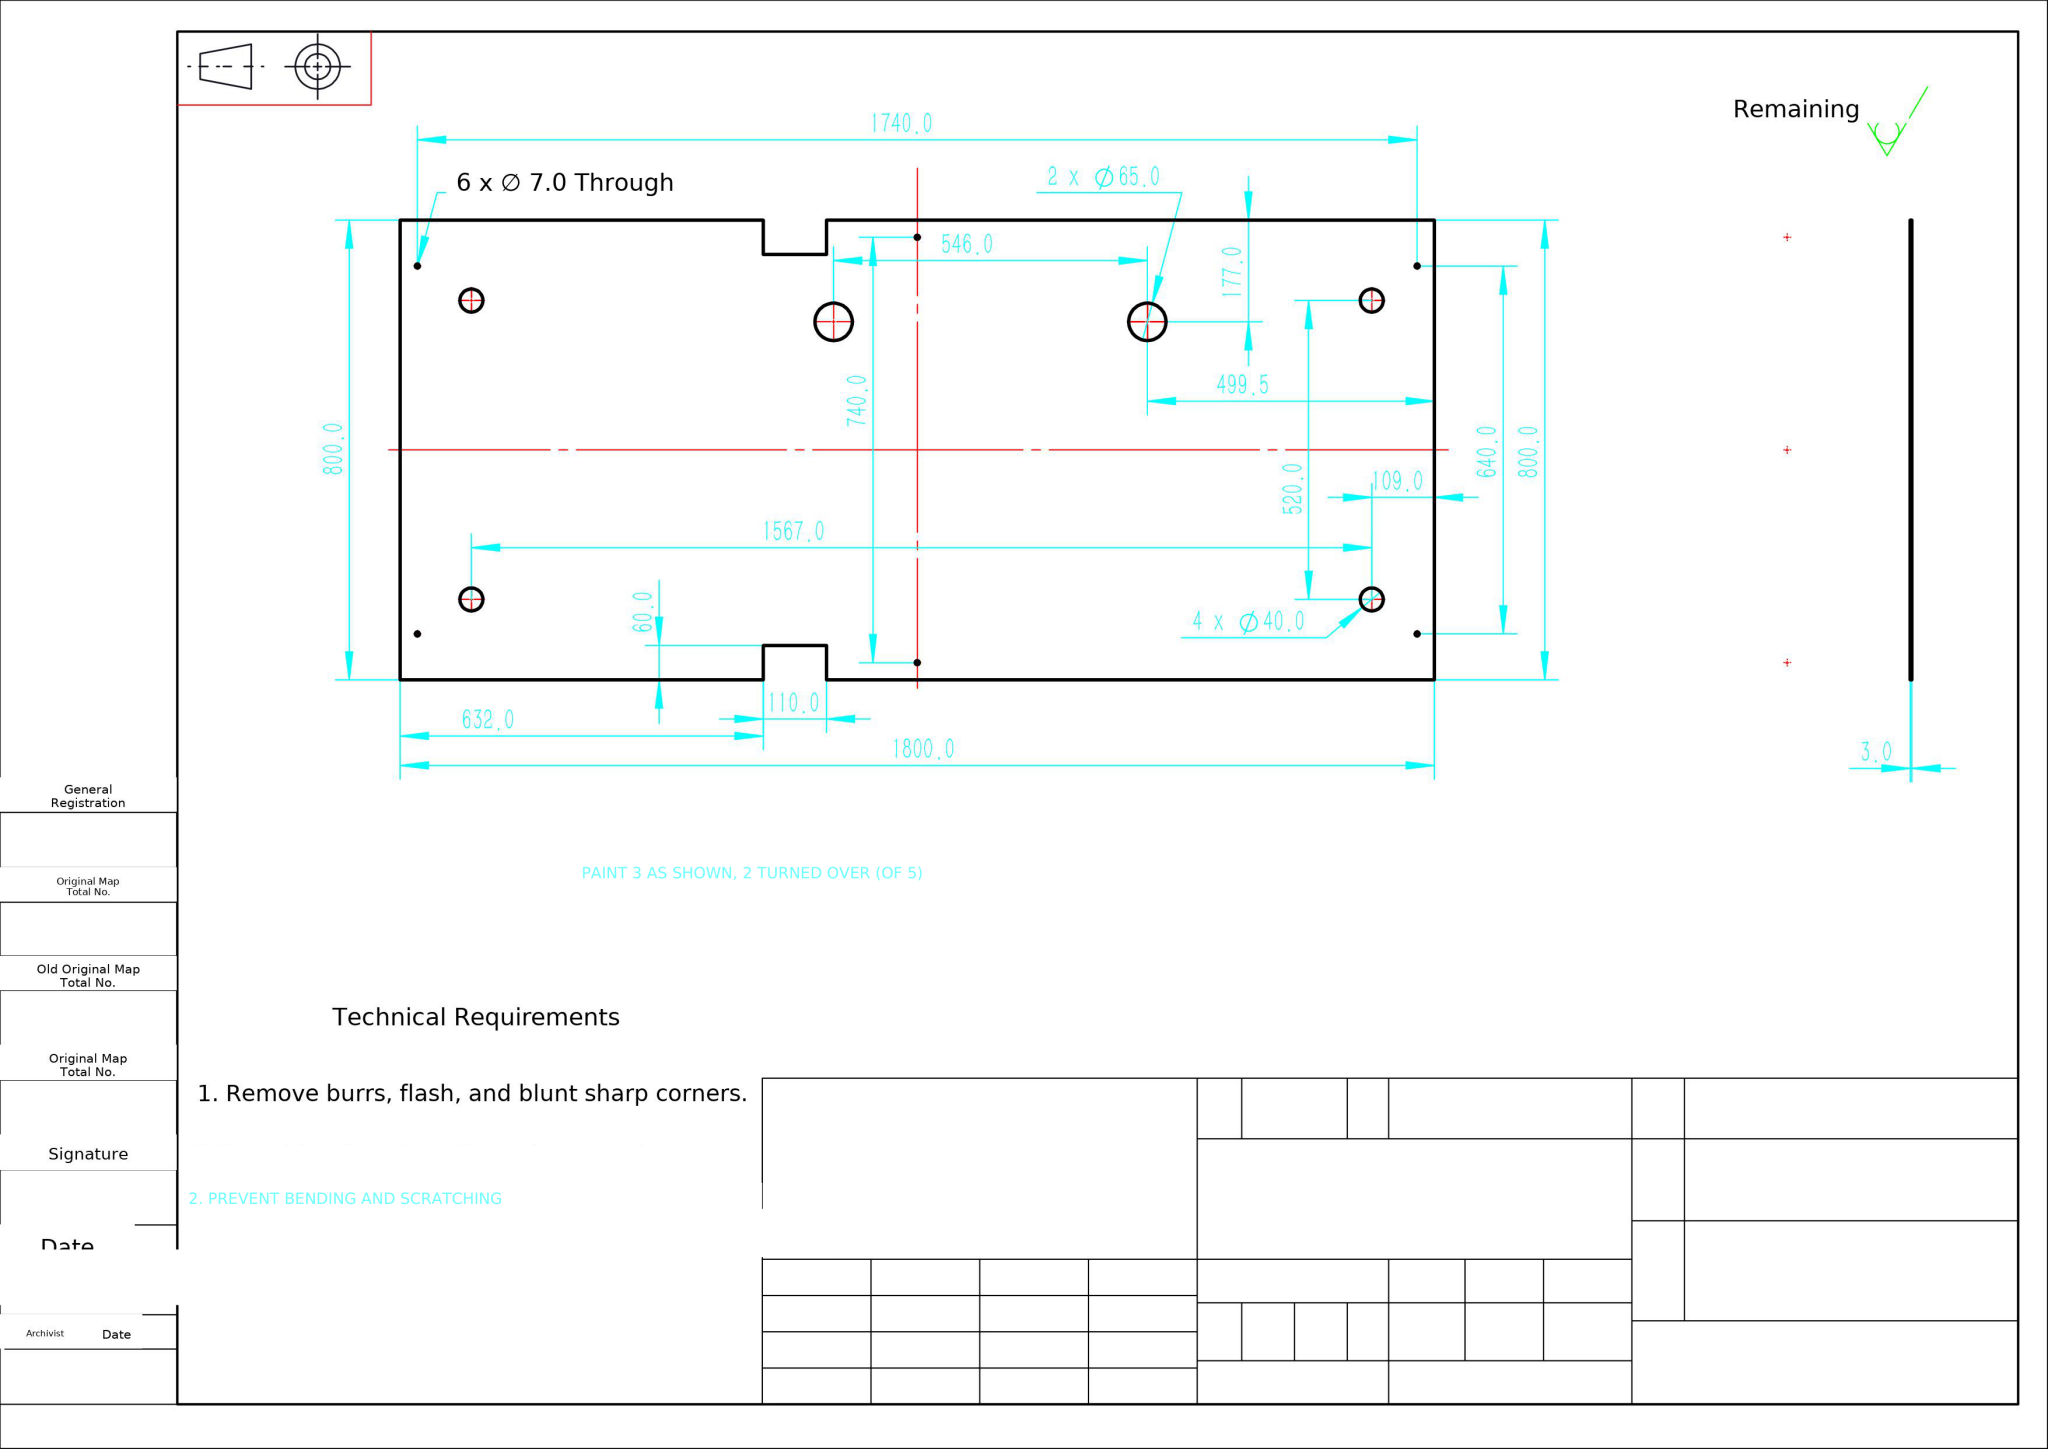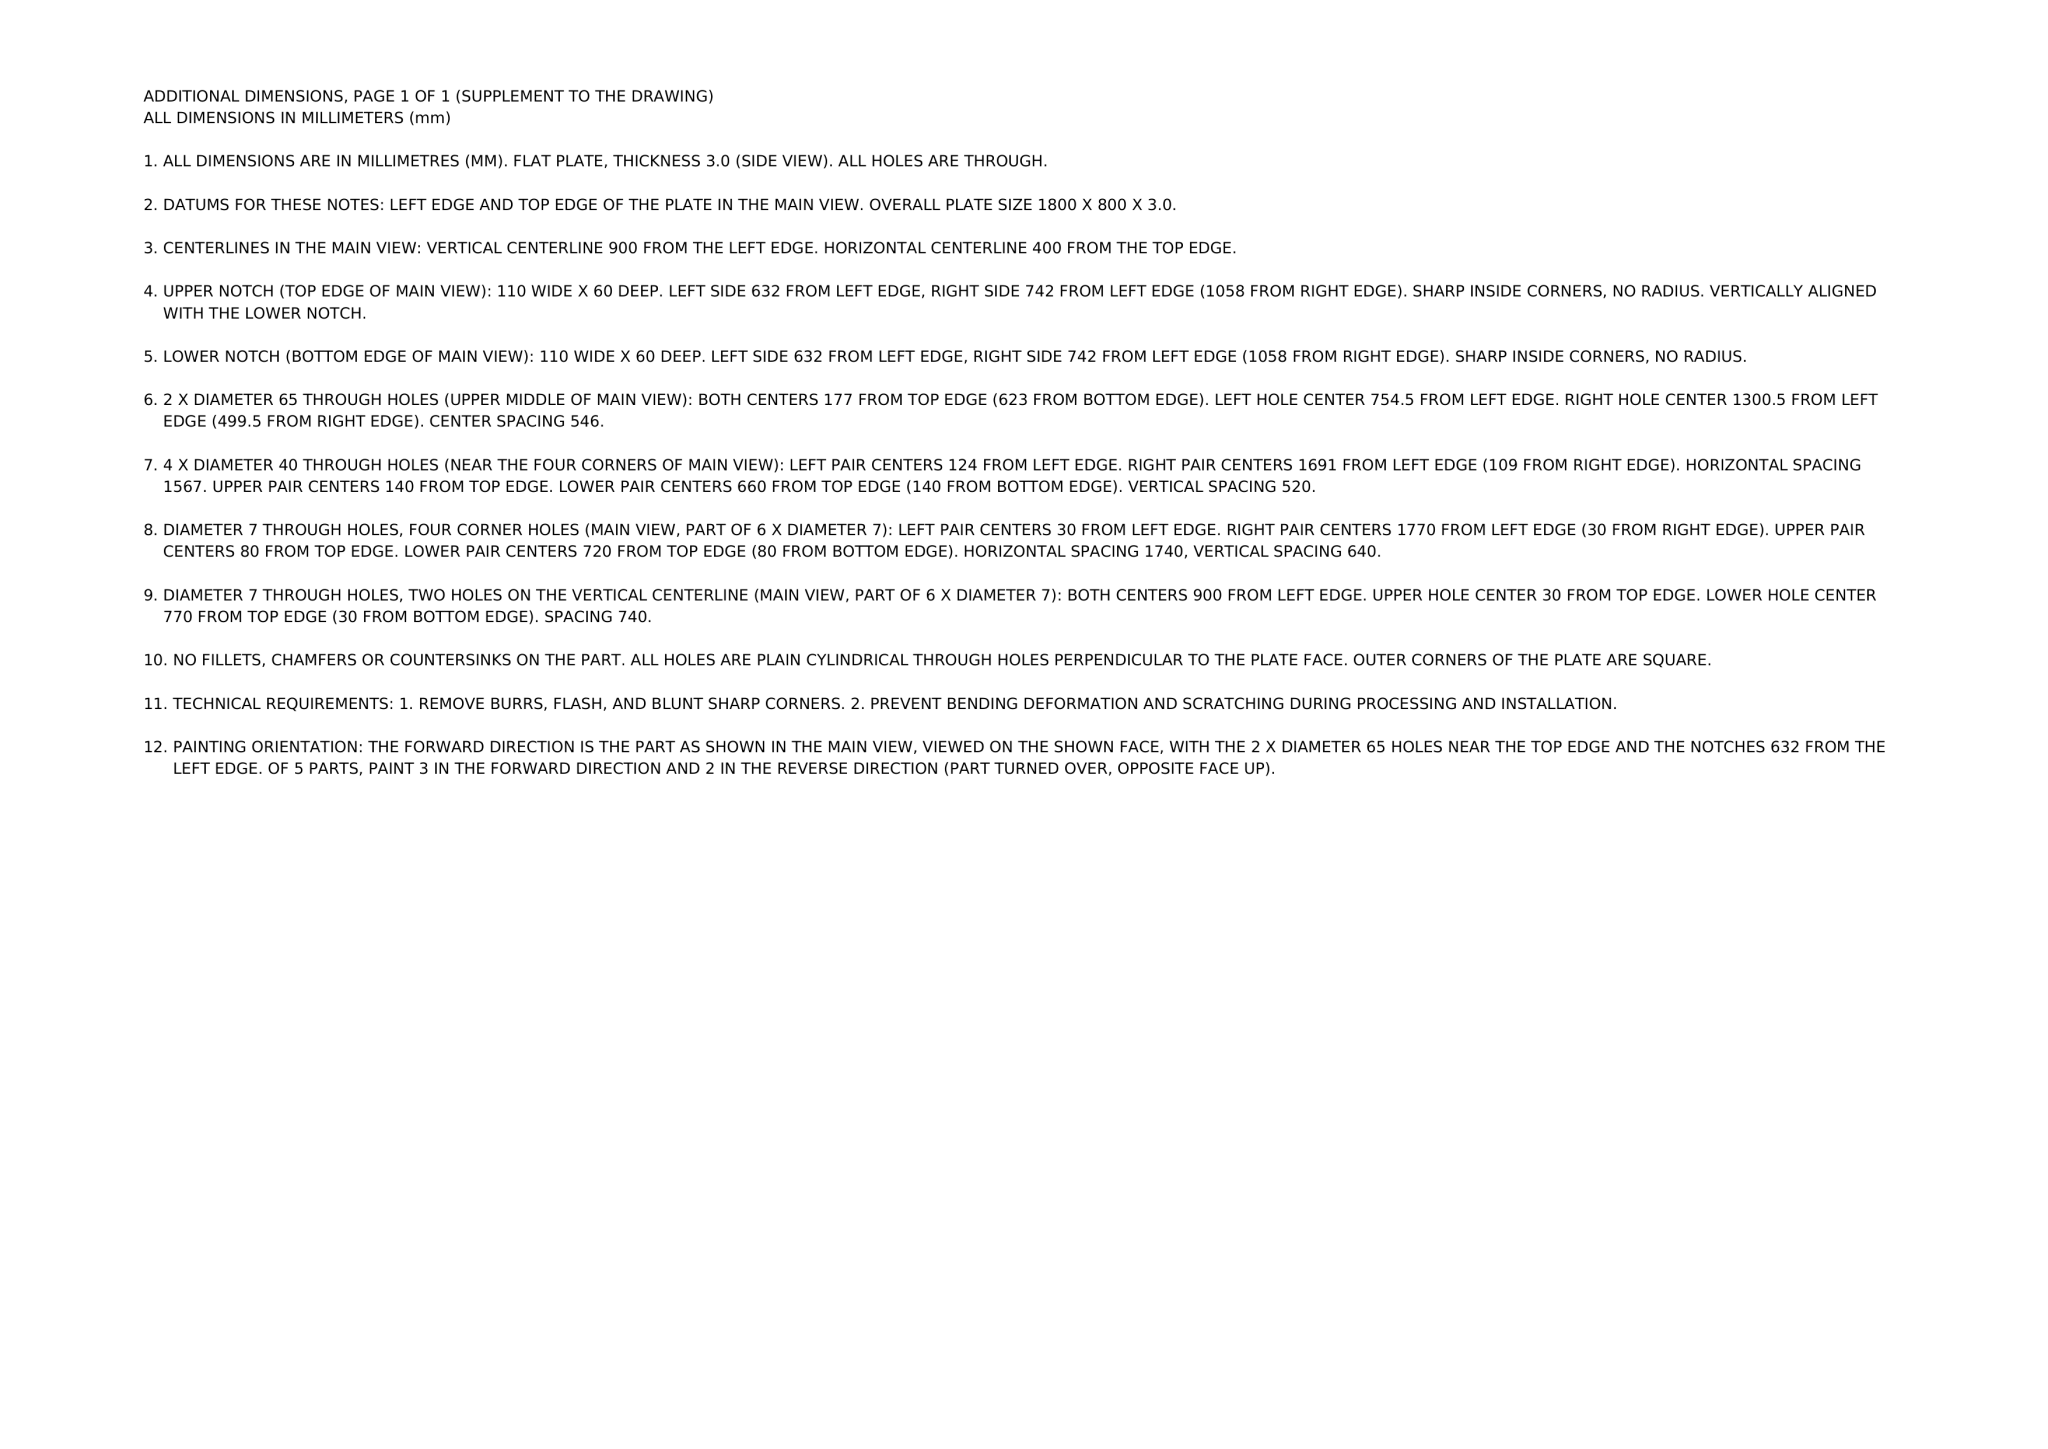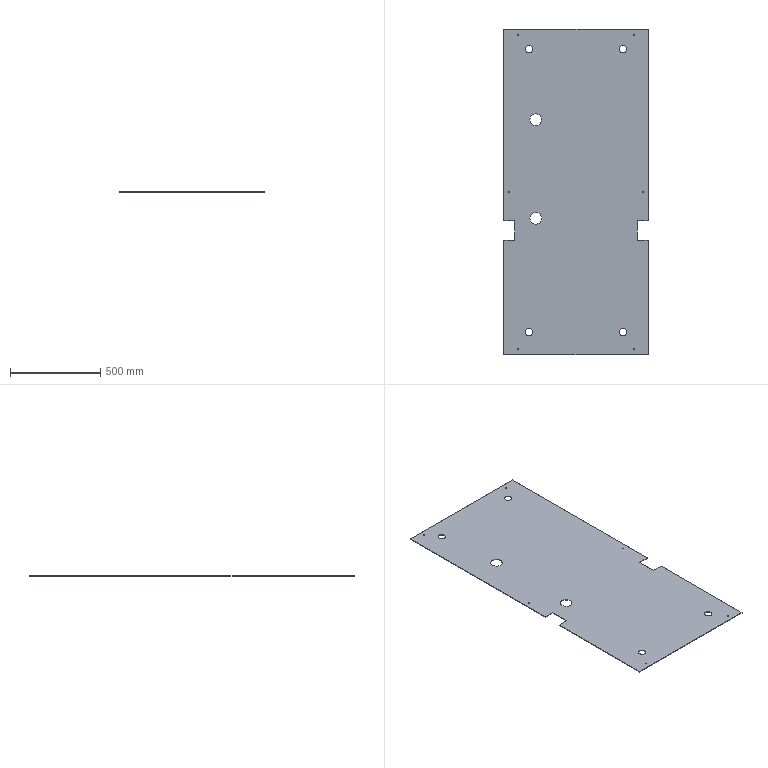Part | NX | mm | 1 solid | 38 faces | box 800 x 1800 x 3 mm | volume 4244718 mm3 | cylinder 24 | plane 14 | commonest cylinder face diameters 7 x12 40 x8 65 x4